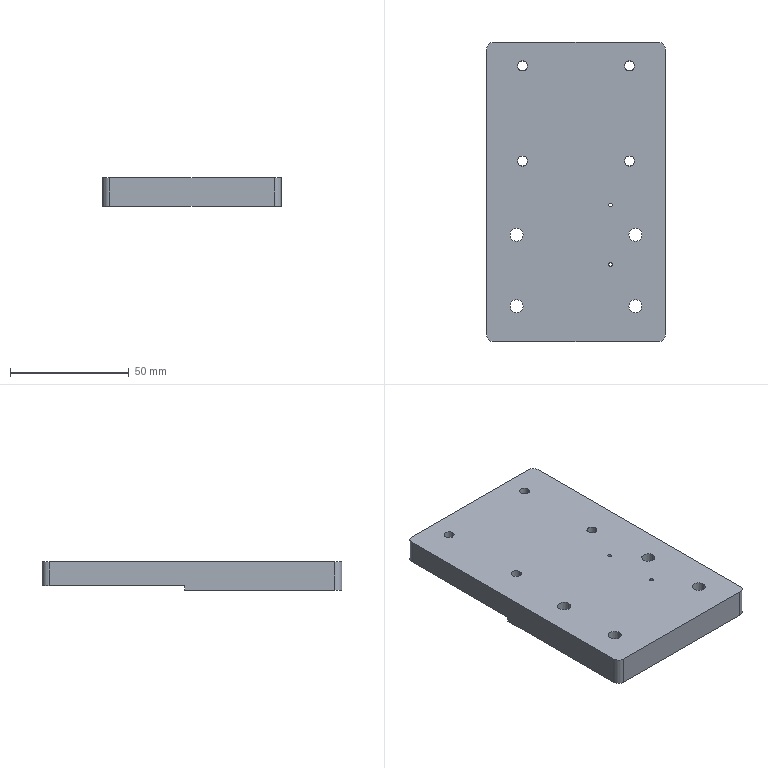CAM job | Mastercam | mm | 13 operations | part box 75 x 126 x 12
1. Facing | 20 - 63 平铣刀
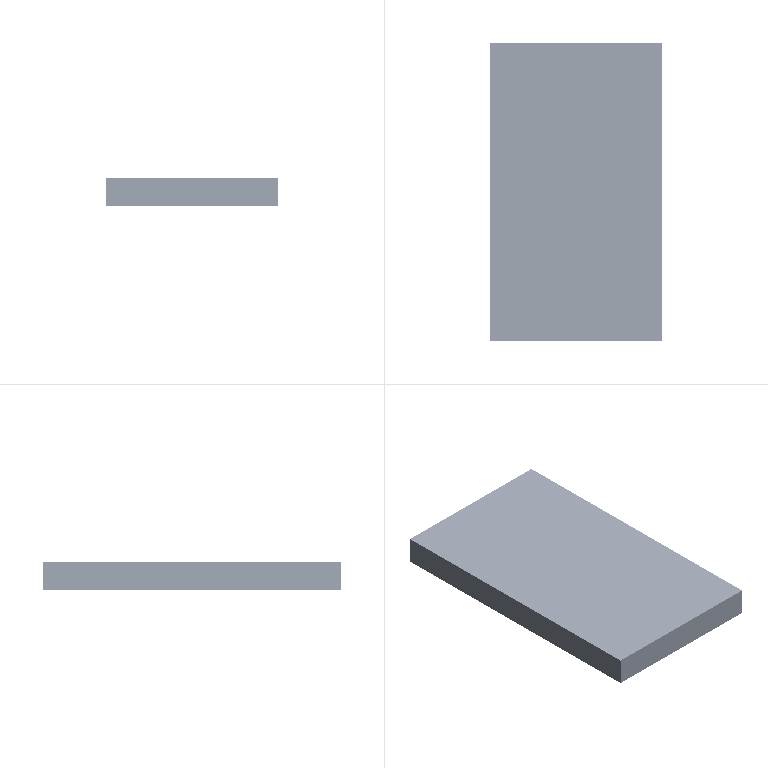2. Contour (Ramp) | 9 - 10 平铣刀
3. Contour (Ramp) | 9 - 10 平铣刀
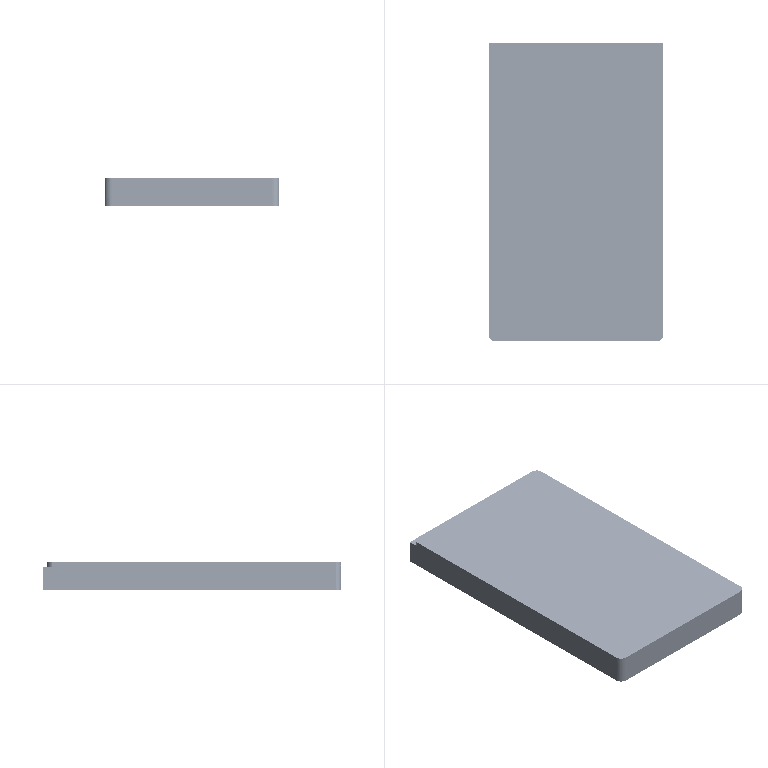4. Contour (2D) | 10 - 10 平铣刀
5. Contour (2D chamfer) | 7 - 4 倒角刀
6. Facing | 20 - 63 平铣刀
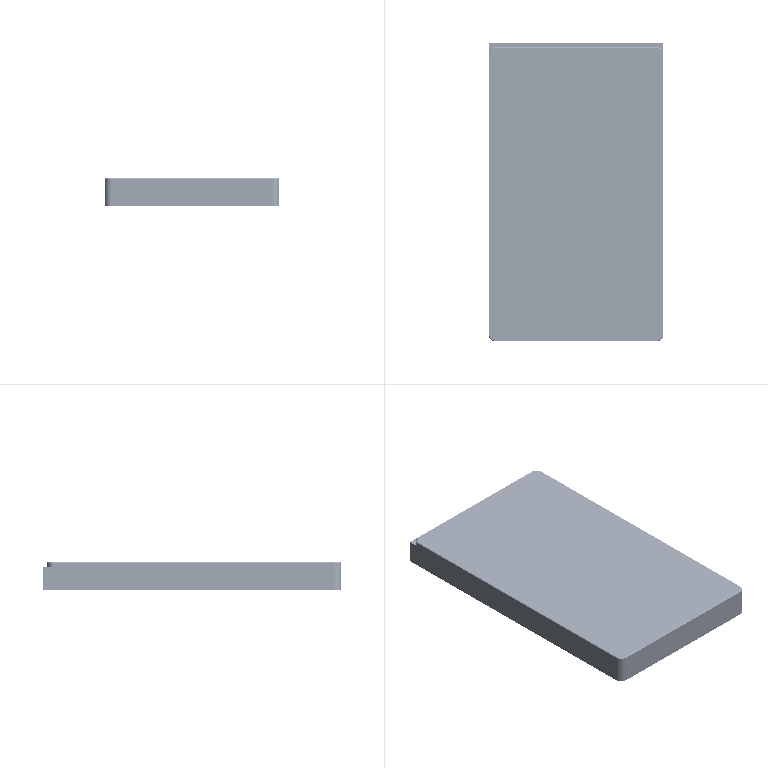7. Contour (Ramp) | 9 - 10 平铣刀
8. Contour (Ramp) | 9 - 10 平铣刀
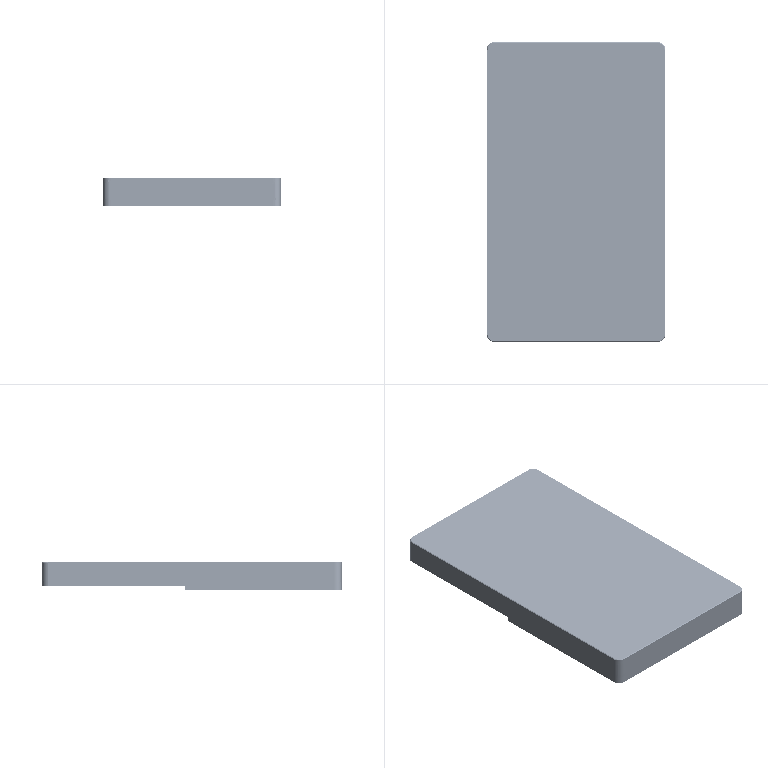9. Contour (2D) | 10 - 10 平铣刀
10. Contour (2D) | 10 - 10 平铣刀
11. Helix Bore | 6 - 6 平铣刀
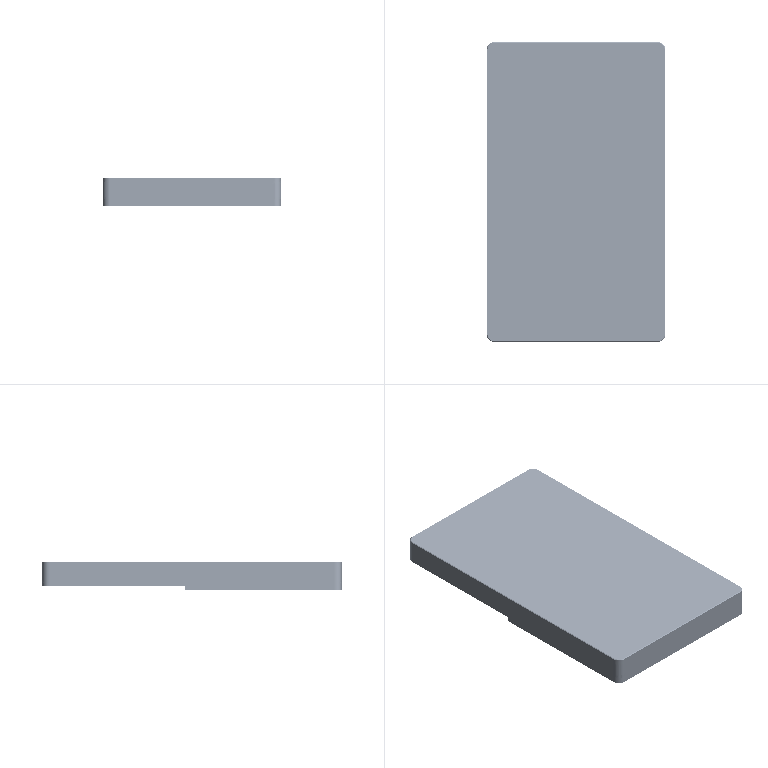12. Drill/Counterbore | 7 - 4 倒角刀
13. Model Chamfer | 7 - 4 倒角刀